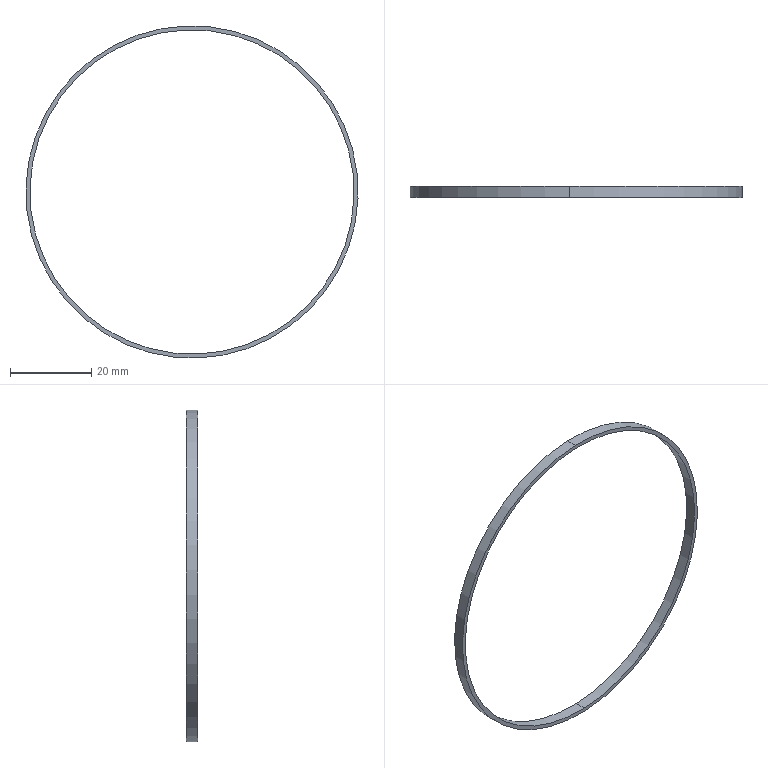Component | SolidWorks | 17-1 | 1 solid | 6 faces | box 82 x 2.75 x 82 mm | volume 700 mm3 | cylinder 4 | plane 2 | commonest cylinder face diameters 80 x2 82 x2
build123d program:
from build123d import *

# Parameters (mm, degrees)
SKETCH1_R           = 41
SKETCH1_R_2         = 40
BOSS_EXTRUDE1_DEPTH = 2.75


with BuildPart() as part:
    # Sketch1 → Boss-Extrude1 (new body)
    with BuildSketch(Plane(origin=(0, 0, 0), x_dir=(1, 0, 0), z_dir=(0, 1, 0))):
        with Locations(Location((0, 0, 0), (0, 0, 270))):
            Circle(SKETCH1_R)
        with Locations(Location((0, 0, 0), (0, 0, 270))):
            Circle(SKETCH1_R_2, mode=Mode.SUBTRACT)
    extrude(amount=BOSS_EXTRUDE1_DEPTH)


solid = part.part

# Placed as in the assembly
solid = solid.moved(Location((0, -23.631, 0), (0, 0, 0)))
STEP:
#1=COLOUR_RGB('',0.7922,0.8196,0.9333);
#2=FILL_AREA_STYLE_COLOUR('',#1);
#3=FILL_AREA_STYLE('',(#2));
#4=SURFACE_STYLE_FILL_AREA(#3);
#5=SURFACE_SIDE_STYLE('',(#4));
#6=SURFACE_STYLE_USAGE(.BOTH.,#5);
#7=PRESENTATION_STYLE_ASSIGNMENT((#6));
#8=CARTESIAN_POINT('',(0.06,-0.8221,-1.574));
#9=VERTEX_POINT('',#8);
#10=CARTESIAN_POINT('',(-0.06,-0.8221,1.574));
#11=VERTEX_POINT('',#10);
#12=CARTESIAN_POINT('',(0.,-0.8221,-0.));
#13=DIRECTION('',(0.,1.,0.));
#14=DIRECTION('',(-0.0381,0.,0.9993));
#15=AXIS2_PLACEMENT_3D('',#12,#13,#14);
#16=CIRCLE('',#15,1.575);
#17=EDGE_CURVE('',#9,#11,#16,.T.);
#18=ORIENTED_EDGE('',*,*,#17,.T.);
#19=CARTESIAN_POINT('',(-0.06,-0.9304,1.574));
#20=VERTEX_POINT('',#19);
#21=CARTESIAN_POINT('',(-0.06,-0.8221,1.574));
#22=DIRECTION('',(0.,-1.,0.));
#23=VECTOR('',#22,39.37);
#24=LINE('',#21,#23);
#25=EDGE_CURVE('',#11,#20,#24,.T.);
#26=ORIENTED_EDGE('',*,*,#25,.T.);
#27=CARTESIAN_POINT('',(0.06,-0.9304,-1.574));
#28=VERTEX_POINT('',#27);
#29=CARTESIAN_POINT('',(0.,-0.9304,-0.));
#30=DIRECTION('',(0.,1.,0.));
#31=DIRECTION('',(-0.0381,0.,0.9993));
#32=AXIS2_PLACEMENT_3D('',#29,#30,#31);
#33=CIRCLE('',#32,1.575);
#34=EDGE_CURVE('',#28,#20,#33,.T.);
#35=ORIENTED_EDGE('',*,*,#34,.F.);
#36=CARTESIAN_POINT('',(0.06,-0.8221,-1.574));
#37=DIRECTION('',(0.,-1.,0.));
#38=VECTOR('',#37,39.37);
#39=LINE('',#36,#38);
#40=EDGE_CURVE('',#9,#28,#39,.T.);
#41=ORIENTED_EDGE('',*,*,#40,.F.);
#42=EDGE_LOOP('',(#18,#26,#35,#41));
#43=FACE_OUTER_BOUND('',#42,.T.);
#44=CARTESIAN_POINT('',(0.,-0.8221,-0.));
#45=DIRECTION('',(0.,-1.,0.));
#46=DIRECTION('',(0.0381,0.,-0.9993));
#47=AXIS2_PLACEMENT_3D('',#44,#45,#46);
#48=CYLINDRICAL_SURFACE('',#47,1.575);
#49=ADVANCED_FACE('',(#43),#48,.F.);
#50=CARTESIAN_POINT('',(-0.0615,-0.8221,1.613));
#51=VERTEX_POINT('',#50);
#52=CARTESIAN_POINT('',(0.0615,-0.8221,-1.613));
#53=VERTEX_POINT('',#52);
#54=CARTESIAN_POINT('',(0.,-0.8221,-0.));
#55=DIRECTION('',(0.,1.,0.));
#56=DIRECTION('',(-0.0381,0.,0.9993));
#57=AXIS2_PLACEMENT_3D('',#54,#55,#56);
#58=CIRCLE('',#57,1.614);
#59=EDGE_CURVE('',#51,#53,#58,.T.);
#60=ORIENTED_EDGE('',*,*,#59,.F.);
#61=CARTESIAN_POINT('',(-0.0615,-0.9304,1.613));
#62=VERTEX_POINT('',#61);
#63=CARTESIAN_POINT('',(-0.0615,-0.8221,1.613));
#64=DIRECTION('',(0.,-1.,0.));
#65=VECTOR('',#64,39.37);
#66=LINE('',#63,#65);
#67=EDGE_CURVE('',#51,#62,#66,.T.);
#68=ORIENTED_EDGE('',*,*,#67,.T.);
#69=CARTESIAN_POINT('',(0.0615,-0.9304,-1.613));
#70=VERTEX_POINT('',#69);
#71=CARTESIAN_POINT('',(0.,-0.9304,-0.));
#72=DIRECTION('',(0.,1.,0.));
#73=DIRECTION('',(-0.0381,0.,0.9993));
#74=AXIS2_PLACEMENT_3D('',#71,#72,#73);
#75=CIRCLE('',#74,1.614);
#76=EDGE_CURVE('',#62,#70,#75,.T.);
#77=ORIENTED_EDGE('',*,*,#76,.T.);
#78=CARTESIAN_POINT('',(0.0615,-0.8221,-1.613));
#79=DIRECTION('',(0.,-1.,0.));
#80=VECTOR('',#79,39.37);
#81=LINE('',#78,#80);
#82=EDGE_CURVE('',#53,#70,#81,.T.);
#83=ORIENTED_EDGE('',*,*,#82,.F.);
#84=EDGE_LOOP('',(#60,#68,#77,#83));
#85=FACE_OUTER_BOUND('',#84,.T.);
#86=CARTESIAN_POINT('',(0.,-0.8221,-0.));
#87=DIRECTION('',(0.,-1.,0.));
#88=DIRECTION('',(0.0381,0.,-0.9993));
#89=AXIS2_PLACEMENT_3D('',#86,#87,#88);
#90=CYLINDRICAL_SURFACE('',#89,1.614);
#91=ADVANCED_FACE('',(#85),#90,.T.);
#92=CARTESIAN_POINT('',(0.,-0.8221,-0.));
#93=DIRECTION('',(0.,1.,0.));
#94=DIRECTION('',(-0.0381,0.,0.9993));
#95=AXIS2_PLACEMENT_3D('',#92,#93,#94);
#96=CIRCLE('',#95,1.614);
#97=EDGE_CURVE('',#53,#51,#96,.T.);
#98=ORIENTED_EDGE('',*,*,#97,.T.);
#99=ORIENTED_EDGE('',*,*,#59,.T.);
#100=EDGE_LOOP('',(#98,#99));
#101=FACE_OUTER_BOUND('',#100,.T.);
#102=ORIENTED_EDGE('',*,*,#17,.F.);
#103=CARTESIAN_POINT('',(0.,-0.8221,-0.));
#104=DIRECTION('',(0.,1.,0.));
#105=DIRECTION('',(-0.0381,0.,0.9993));
#106=AXIS2_PLACEMENT_3D('',#103,#104,#105);
#107=CIRCLE('',#106,1.575);
#108=EDGE_CURVE('',#11,#9,#107,.T.);
#109=ORIENTED_EDGE('',*,*,#108,.F.);
#110=EDGE_LOOP('',(#102,#109));
#111=FACE_BOUND('',#110,.T.);
#112=CARTESIAN_POINT('',(0.,-0.8221,-0.));
#113=DIRECTION('',(0.,1.,0.));
#114=DIRECTION('',(-0.0381,0.,0.9993));
#115=AXIS2_PLACEMENT_3D('',#112,#113,#114);
#116=PLANE('',#115);
#117=ADVANCED_FACE('',(#101,#111),#116,.T.);
#118=CARTESIAN_POINT('',(0.,-0.9304,-0.));
#119=DIRECTION('',(0.,1.,0.));
#120=DIRECTION('',(-0.0381,0.,0.9993));
#121=AXIS2_PLACEMENT_3D('',#118,#119,#120);
#122=CIRCLE('',#121,1.614);
#123=EDGE_CURVE('',#70,#62,#122,.T.);
#124=ORIENTED_EDGE('',*,*,#123,.F.);
#125=ORIENTED_EDGE('',*,*,#76,.F.);
#126=EDGE_LOOP('',(#124,#125));
#127=FACE_OUTER_BOUND('',#126,.T.);
#128=ORIENTED_EDGE('',*,*,#34,.T.);
#129=CARTESIAN_POINT('',(0.,-0.9304,-0.));
#130=DIRECTION('',(0.,1.,0.));
#131=DIRECTION('',(-0.0381,0.,0.9993));
#132=AXIS2_PLACEMENT_3D('',#129,#130,#131);
#133=CIRCLE('',#132,1.575);
#134=EDGE_CURVE('',#20,#28,#133,.T.);
#135=ORIENTED_EDGE('',*,*,#134,.T.);
#136=EDGE_LOOP('',(#128,#135));
#137=FACE_BOUND('',#136,.T.);
#138=CARTESIAN_POINT('',(0.,-0.9304,-0.));
#139=DIRECTION('',(0.,1.,0.));
#140=DIRECTION('',(-0.0381,0.,0.9993));
#141=AXIS2_PLACEMENT_3D('',#138,#139,#140);
#142=PLANE('',#141);
#143=ADVANCED_FACE('',(#127,#137),#142,.F.);
#144=ORIENTED_EDGE('',*,*,#67,.F.);
#145=ORIENTED_EDGE('',*,*,#97,.F.);
#146=ORIENTED_EDGE('',*,*,#82,.T.);
#147=ORIENTED_EDGE('',*,*,#123,.T.);
#148=EDGE_LOOP('',(#144,#145,#146,#147));
#149=FACE_OUTER_BOUND('',#148,.T.);
#150=CARTESIAN_POINT('',(0.,-0.8221,-0.));
#151=DIRECTION('',(0.,-1.,0.));
#152=DIRECTION('',(0.0381,0.,-0.9993));
#153=AXIS2_PLACEMENT_3D('',#150,#151,#152);
#154=CYLINDRICAL_SURFACE('',#153,1.614);
#155=ADVANCED_FACE('',(#149),#154,.T.);
#156=ORIENTED_EDGE('',*,*,#25,.F.);
#157=ORIENTED_EDGE('',*,*,#108,.T.);
#158=ORIENTED_EDGE('',*,*,#40,.T.);
#159=ORIENTED_EDGE('',*,*,#134,.F.);
#160=EDGE_LOOP('',(#156,#157,#158,#159));
#161=FACE_OUTER_BOUND('',#160,.T.);
#162=CARTESIAN_POINT('',(0.,-0.8221,-0.));
#163=DIRECTION('',(0.,-1.,0.));
#164=DIRECTION('',(0.0381,0.,-0.9993));
#165=AXIS2_PLACEMENT_3D('',#162,#163,#164);
#166=CYLINDRICAL_SURFACE('',#165,1.575);
#167=ADVANCED_FACE('',(#161),#166,.F.);
#168=CLOSED_SHELL('',(#49,#91,#117,#143,#155,#167));
#169=MANIFOLD_SOLID_BREP('',#168);
#170=STYLED_ITEM('',(#7),#169);
#171=(LENGTH_UNIT()NAMED_UNIT(*)SI_UNIT($,.METRE.));
#172=LENGTH_MEASURE_WITH_UNIT(LENGTH_MEASURE(0.0254),#171);
#173=DIMENSIONAL_EXPONENTS(1.,0.,0.,0.,0.,0.,0.);
#174=(CONVERSION_BASED_UNIT('',#172)LENGTH_UNIT()NAMED_UNIT(#173));
#175=UNCERTAINTY_MEASURE_WITH_UNIT(LENGTH_MEASURE(0.00001),#174,'','');
#176=(NAMED_UNIT(*)PLANE_ANGLE_UNIT()SI_UNIT($,.RADIAN.));
#177=(NAMED_UNIT(*)SI_UNIT($,.STERADIAN.)SOLID_ANGLE_UNIT());
#178=(GEOMETRIC_REPRESENTATION_CONTEXT(3)GLOBAL_UNCERTAINTY_ASSIGNED_CONTEXT((#175))GLOBAL_UNIT_ASSIGNED_CONTEXT((#174,#176,#177))REPRESENTATION_CONTEXT('',''));
#179=MECHANICAL_DESIGN_GEOMETRIC_PRESENTATION_REPRESENTATION('',(#170),#178);
#180=PRESENTATION_LAYER_ASSIGNMENT('','',(#170));
#181=CARTESIAN_POINT('',(0.,0.,0.));
#182=DIRECTION('',(0.,0.,1.));
#183=DIRECTION('',(1.,0.,0.));
#184=AXIS2_PLACEMENT_3D('',#181,#182,#183);
#185=(LENGTH_UNIT()NAMED_UNIT(*)SI_UNIT($,.METRE.));
#186=LENGTH_MEASURE_WITH_UNIT(LENGTH_MEASURE(0.0254),#185);
#187=DIMENSIONAL_EXPONENTS(1.,0.,0.,0.,0.,0.,0.);
#188=(CONVERSION_BASED_UNIT('',#186)LENGTH_UNIT()NAMED_UNIT(#187));
#189=UNCERTAINTY_MEASURE_WITH_UNIT(LENGTH_MEASURE(0.00001),#188,'','');
#190=(NAMED_UNIT(*)PLANE_ANGLE_UNIT()SI_UNIT($,.RADIAN.));
#191=(NAMED_UNIT(*)SI_UNIT($,.STERADIAN.)SOLID_ANGLE_UNIT());
#192=(GEOMETRIC_REPRESENTATION_CONTEXT(3)GLOBAL_UNCERTAINTY_ASSIGNED_CONTEXT((#189))GLOBAL_UNIT_ASSIGNED_CONTEXT((#188,#190,#191))REPRESENTATION_CONTEXT('',''));
#193=ADVANCED_BREP_SHAPE_REPRESENTATION('',(#169,#184),#192);